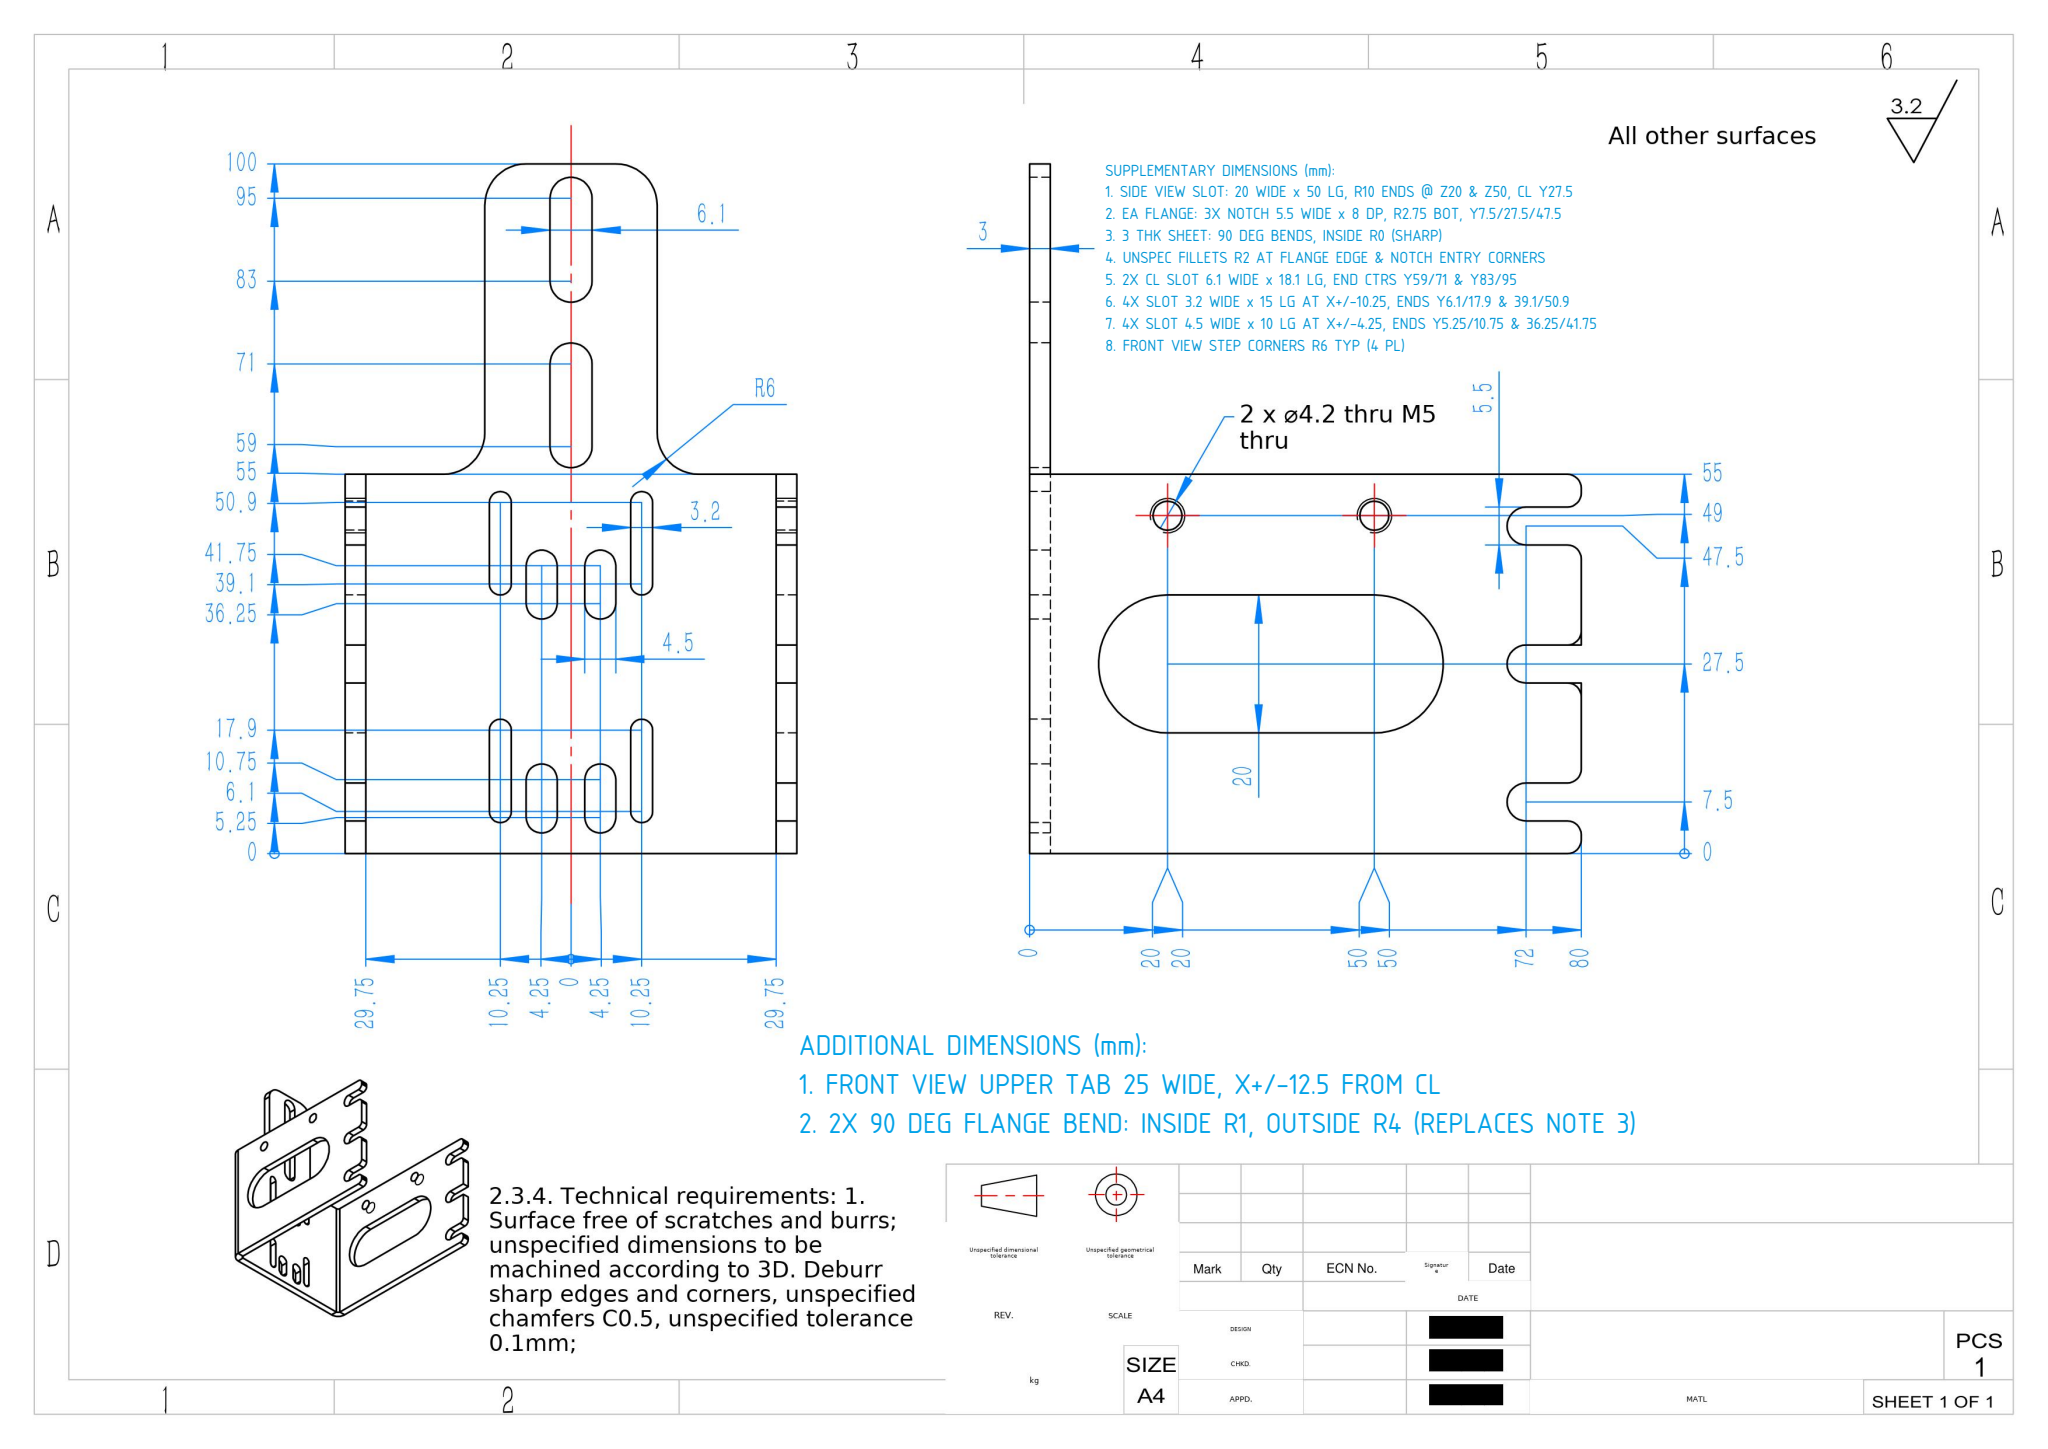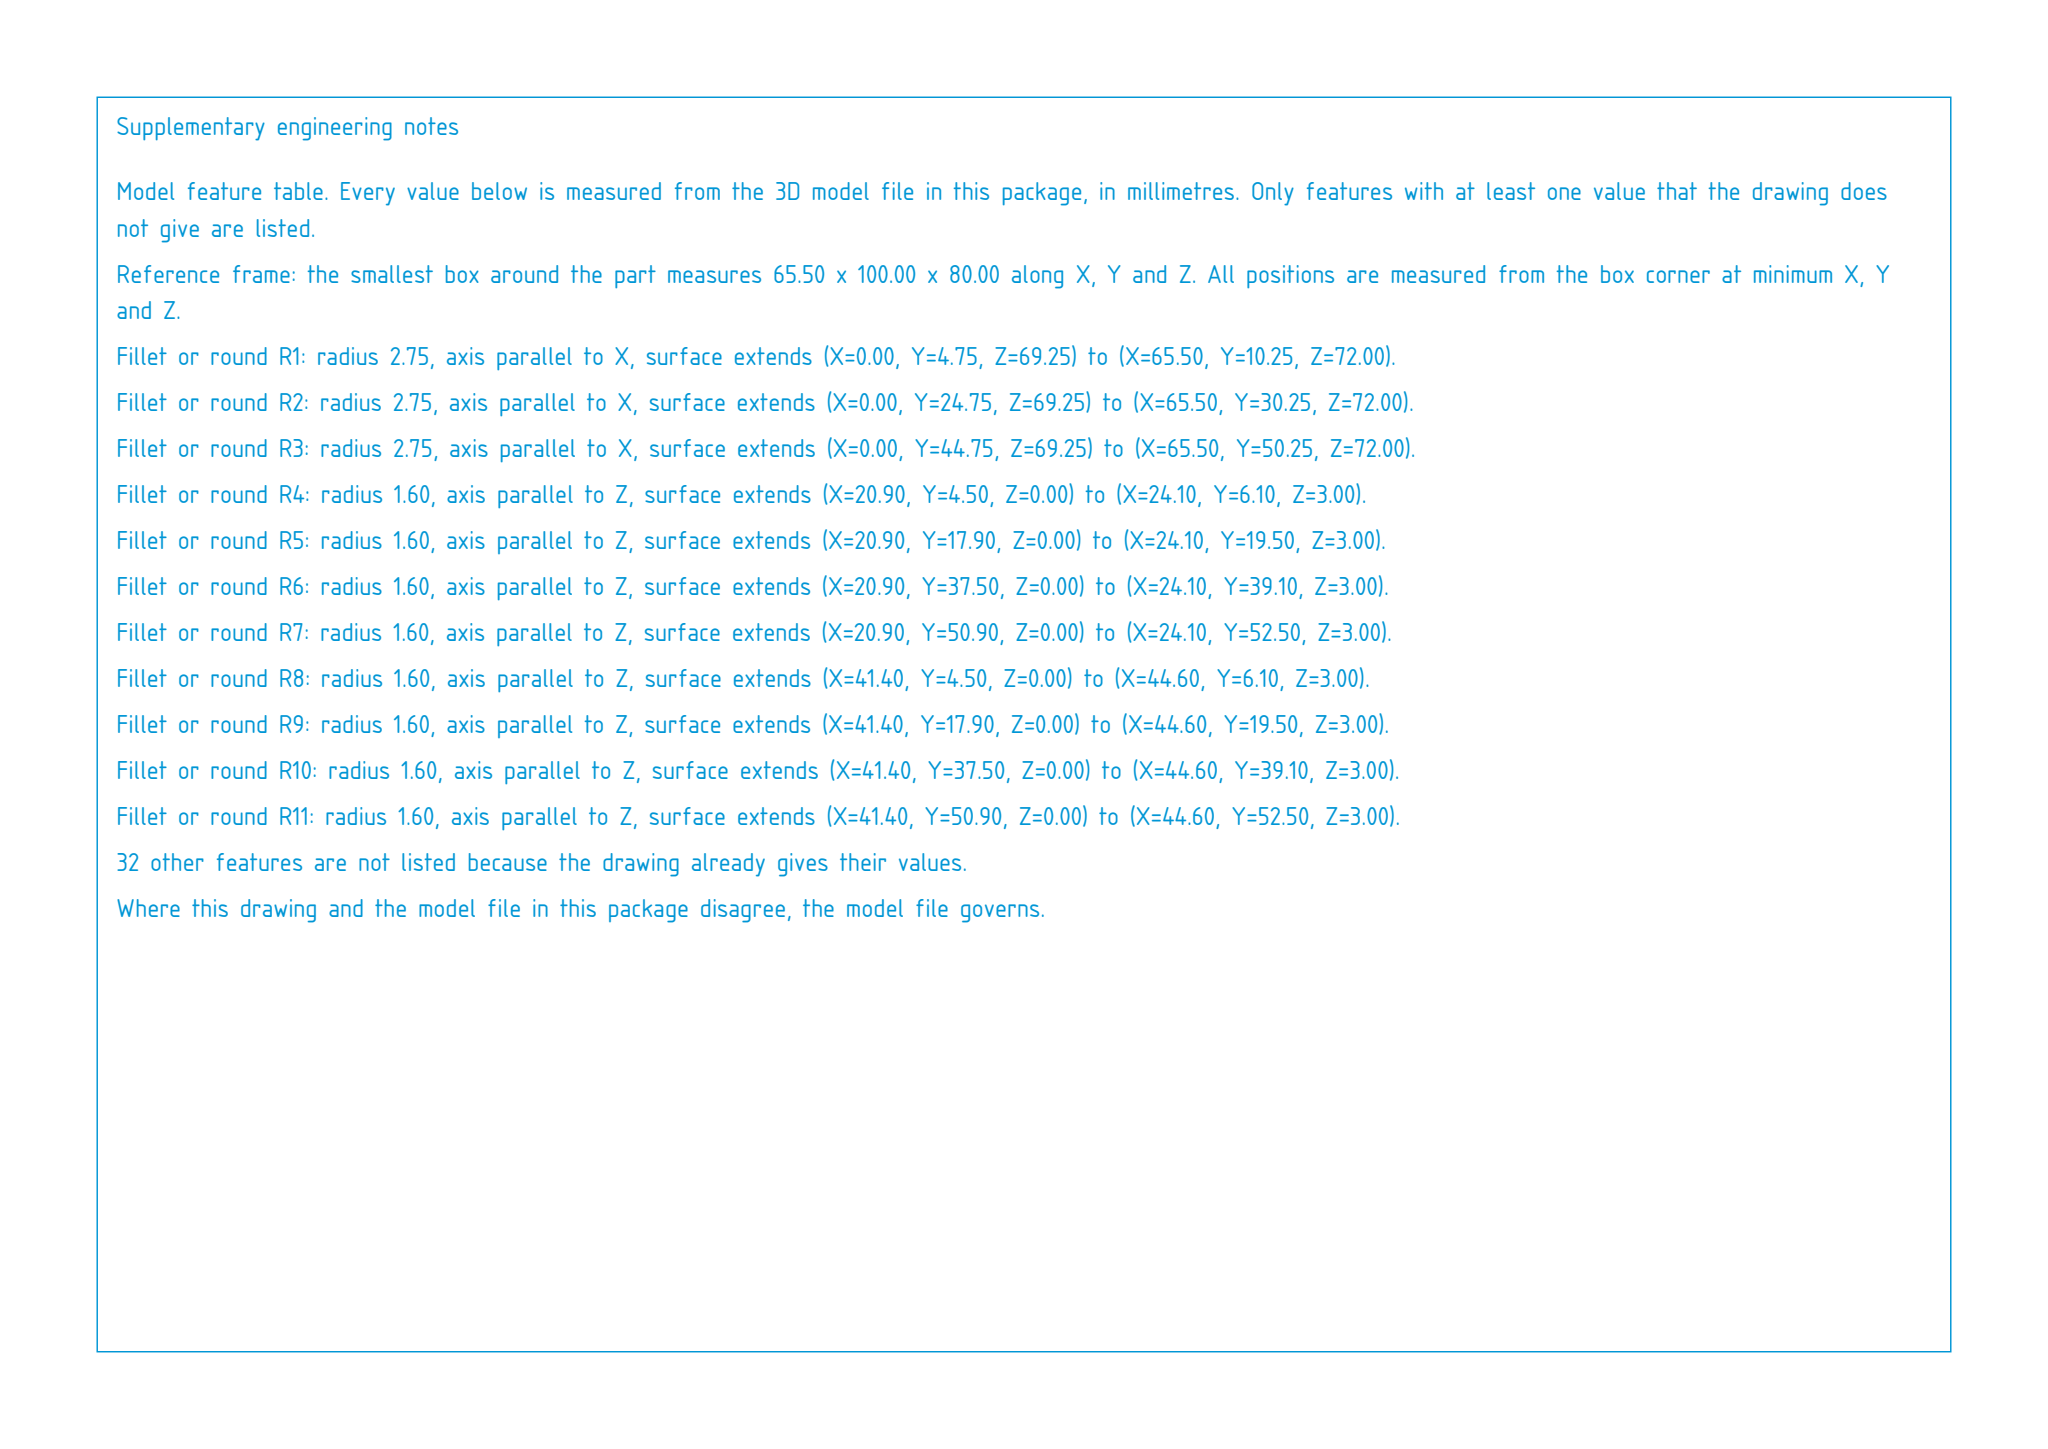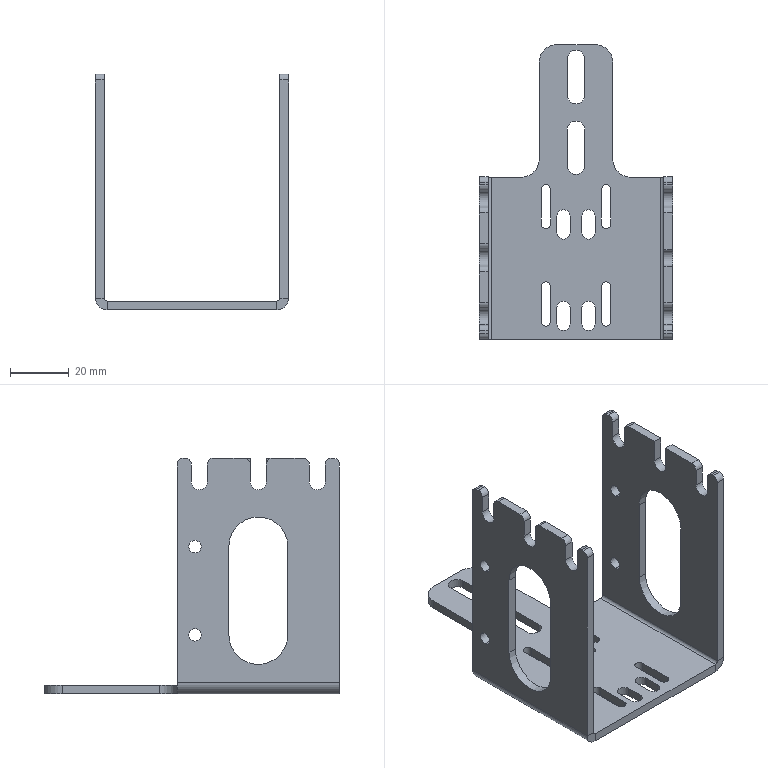Part | SolidWorks | mm | 1 solid | 126 faces | box 65.5 x 100 x 80 mm | volume 30893 mm3 | plane 64 | cylinder 62 | commonest cylinder face diameters 4 x14 4.2 x8 3.2 x8 4.5 x8 20 x6 5.5 x6 6.1 x4 12 x4